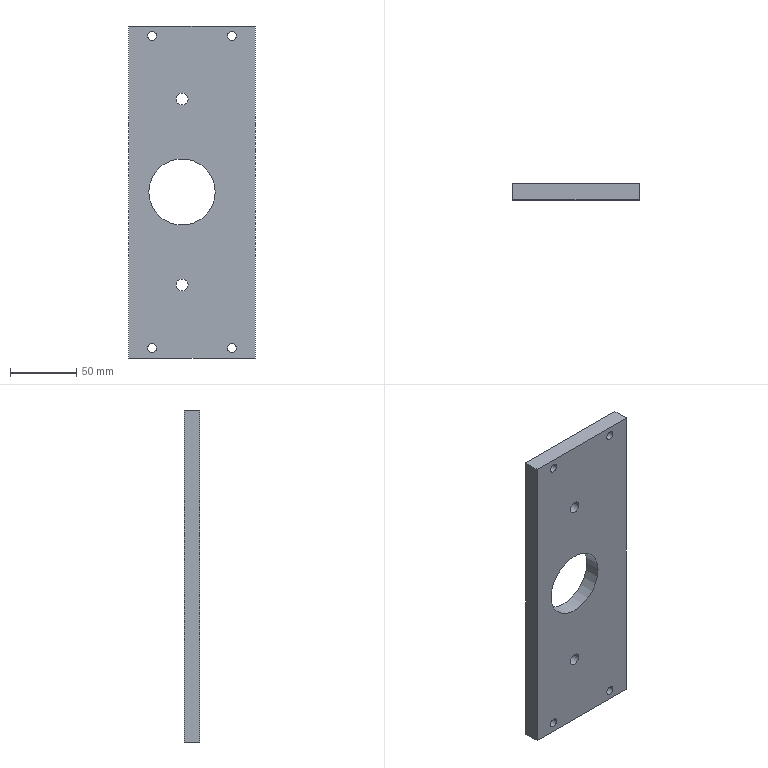Component | SolidWorks | 8TC-A15004-D0-03A-1 | 1 solid | 32 faces | box 95 x 12 x 250 mm | volume 256712 mm3 | cylinder 22 | plane 10 | commonest cylinder face diameters 11 x8 6.6 x8 9 x4 50 x2 | material #45
build123d program:
from build123d import *

# Parameters (mm, degrees)
SKETCH1_W                                       = 250
SKETCH1_H                                       = 95
BOSS_EXTRUDE1_DEPTH                             = 6
M8_CLEARANCE_HOLE_2_D                           = 9
M8_CLEARANCE_HOLE_1_D                           = 50
M6_HEX_SOCKET_HEAD_CAP_SCREW_CBORE1_D           = 6.6
M6_HEX_SOCKET_HEAD_CAP_SCREW_CBORE1_CBORE_D     = 11
M6_HEX_SOCKET_HEAD_CAP_SCREW_CBORE1_CBORE_DEPTH = 6.4


with BuildPart() as part:
    # Sketch1 → Boss-Extrude1 (new, symmetric)
    with BuildSketch(Plane(origin=(0, 0, 0), x_dir=(1, 0, 0), z_dir=(0, 1, 0))):
        Rectangle(SKETCH1_W, SKETCH1_H)
    extrude(amount=BOSS_EXTRUDE1_DEPTH, both=True)

    # M8 Clearance Hole 2 (through all)
    with Locations(Plane(origin=(0, -6, 0), x_dir=(-1, 0, 0), z_dir=(0, -1, 0))):
        with Locations((-70, -7.5), (70, -7.5)):
            Hole(M8_CLEARANCE_HOLE_2_D / 2)

    # M8 Clearance Hole 1 (through all)
    with Locations(Plane(origin=(0, -6, 0), x_dir=(-1, 0, 0), z_dir=(0, -1, 0))):
        with Locations((0, -7.5)):
            Hole(M8_CLEARANCE_HOLE_1_D / 2)

    # M6 Hex Socket Head Cap Screw CBORE1 (through all)
    with Locations(Plane(origin=(0, -6, 0), x_dir=(-1, 0, 0), z_dir=(0, -1, 0))):
        with Locations((-117.5, 30), (-117.5, -30), (117.5, 30), (117.5, -30)):
            CounterBoreHole(M6_HEX_SOCKET_HEAD_CAP_SCREW_CBORE1_D / 2, M6_HEX_SOCKET_HEAD_CAP_SCREW_CBORE1_CBORE_D / 2, M6_HEX_SOCKET_HEAD_CAP_SCREW_CBORE1_CBORE_DEPTH)


solid = part.part

# Placed as in the assembly
solid = solid.moved(Location((0, 428.5, 0), (180, -90, 0)))
STEP:
#1=CARTESIAN_POINT('',(0.9646,16.854,-4.626));
#2=VERTEX_POINT('',#1);
#3=CARTESIAN_POINT('',(1.398,16.854,-4.626));
#4=VERTEX_POINT('',#3);
#5=CARTESIAN_POINT('',(1.181,16.854,-4.626));
#6=DIRECTION('',(0.,1.,0.));
#7=DIRECTION('',(1.,0.,0.));
#8=AXIS2_PLACEMENT_3D('',#5,#6,#7);
#9=CIRCLE('',#8,0.2165);
#10=EDGE_CURVE('',#2,#4,#9,.T.);
#11=ORIENTED_EDGE('',*,*,#10,.F.);
#12=CARTESIAN_POINT('',(0.9646,17.106,-4.626));
#13=VERTEX_POINT('',#12);
#14=CARTESIAN_POINT('',(0.9646,17.106,-4.626));
#15=DIRECTION('',(0.,1.,0.));
#16=VECTOR('',#15,39.37);
#17=LINE('',#14,#16);
#18=EDGE_CURVE('',#2,#13,#17,.T.);
#19=ORIENTED_EDGE('',*,*,#18,.T.);
#20=CARTESIAN_POINT('',(1.398,17.106,-4.626));
#21=VERTEX_POINT('',#20);
#22=CARTESIAN_POINT('',(1.181,17.106,-4.626));
#23=DIRECTION('',(0.,1.,0.));
#24=DIRECTION('',(1.,0.,0.));
#25=AXIS2_PLACEMENT_3D('',#22,#23,#24);
#26=CIRCLE('',#25,0.2165);
#27=EDGE_CURVE('',#13,#21,#26,.T.);
#28=ORIENTED_EDGE('',*,*,#27,.T.);
#29=CARTESIAN_POINT('',(1.398,17.106,-4.626));
#30=DIRECTION('',(0.,1.,0.));
#31=VECTOR('',#30,39.37);
#32=LINE('',#29,#31);
#33=EDGE_CURVE('',#4,#21,#32,.T.);
#34=ORIENTED_EDGE('',*,*,#33,.F.);
#35=EDGE_LOOP('',(#11,#19,#28,#34));
#36=FACE_OUTER_BOUND('',#35,.T.);
#37=CARTESIAN_POINT('',(1.181,17.106,-4.626));
#38=DIRECTION('',(0.,1.,0.));
#39=DIRECTION('',(1.,0.,0.));
#40=AXIS2_PLACEMENT_3D('',#37,#38,#39);
#41=CYLINDRICAL_SURFACE('',#40,0.2165);
#42=ADVANCED_FACE('',(#36),#41,.F.);
#43=CARTESIAN_POINT('',(1.051,16.634,-4.626));
#44=VERTEX_POINT('',#43);
#45=CARTESIAN_POINT('',(1.311,16.634,-4.626));
#46=VERTEX_POINT('',#45);
#47=CARTESIAN_POINT('',(1.181,16.634,-4.626));
#48=DIRECTION('',(0.,1.,0.));
#49=DIRECTION('',(1.,0.,0.));
#50=AXIS2_PLACEMENT_3D('',#47,#48,#49);
#51=CIRCLE('',#50,0.1299);
#52=EDGE_CURVE('',#44,#46,#51,.T.);
#53=ORIENTED_EDGE('',*,*,#52,.F.);
#54=CARTESIAN_POINT('',(1.051,16.854,-4.626));
#55=VERTEX_POINT('',#54);
#56=CARTESIAN_POINT('',(1.051,17.106,-4.626));
#57=DIRECTION('',(0.,1.,0.));
#58=VECTOR('',#57,39.37);
#59=LINE('',#56,#58);
#60=EDGE_CURVE('',#44,#55,#59,.T.);
#61=ORIENTED_EDGE('',*,*,#60,.T.);
#62=CARTESIAN_POINT('',(1.311,16.854,-4.626));
#63=VERTEX_POINT('',#62);
#64=CARTESIAN_POINT('',(1.181,16.854,-4.626));
#65=DIRECTION('',(0.,1.,0.));
#66=DIRECTION('',(1.,0.,0.));
#67=AXIS2_PLACEMENT_3D('',#64,#65,#66);
#68=CIRCLE('',#67,0.1299);
#69=EDGE_CURVE('',#55,#63,#68,.T.);
#70=ORIENTED_EDGE('',*,*,#69,.T.);
#71=CARTESIAN_POINT('',(1.311,17.106,-4.626));
#72=DIRECTION('',(0.,1.,0.));
#73=VECTOR('',#72,39.37);
#74=LINE('',#71,#73);
#75=EDGE_CURVE('',#46,#63,#74,.T.);
#76=ORIENTED_EDGE('',*,*,#75,.F.);
#77=EDGE_LOOP('',(#53,#61,#70,#76));
#78=FACE_OUTER_BOUND('',#77,.T.);
#79=CARTESIAN_POINT('',(1.181,17.106,-4.626));
#80=DIRECTION('',(0.,1.,0.));
#81=DIRECTION('',(1.,0.,0.));
#82=AXIS2_PLACEMENT_3D('',#79,#80,#81);
#83=CYLINDRICAL_SURFACE('',#82,0.1299);
#84=ADVANCED_FACE('',(#78),#83,.F.);
#85=CARTESIAN_POINT('',(-1.398,16.854,-4.626));
#86=VERTEX_POINT('',#85);
#87=CARTESIAN_POINT('',(-0.9646,16.854,-4.626));
#88=VERTEX_POINT('',#87);
#89=CARTESIAN_POINT('',(-1.181,16.854,-4.626));
#90=DIRECTION('',(0.,1.,0.));
#91=DIRECTION('',(1.,0.,0.));
#92=AXIS2_PLACEMENT_3D('',#89,#90,#91);
#93=CIRCLE('',#92,0.2165);
#94=EDGE_CURVE('',#86,#88,#93,.T.);
#95=ORIENTED_EDGE('',*,*,#94,.F.);
#96=CARTESIAN_POINT('',(-1.398,17.106,-4.626));
#97=VERTEX_POINT('',#96);
#98=CARTESIAN_POINT('',(-1.398,17.106,-4.626));
#99=DIRECTION('',(0.,1.,0.));
#100=VECTOR('',#99,39.37);
#101=LINE('',#98,#100);
#102=EDGE_CURVE('',#86,#97,#101,.T.);
#103=ORIENTED_EDGE('',*,*,#102,.T.);
#104=CARTESIAN_POINT('',(-0.9646,17.106,-4.626));
#105=VERTEX_POINT('',#104);
#106=CARTESIAN_POINT('',(-1.181,17.106,-4.626));
#107=DIRECTION('',(0.,1.,0.));
#108=DIRECTION('',(1.,0.,0.));
#109=AXIS2_PLACEMENT_3D('',#106,#107,#108);
#110=CIRCLE('',#109,0.2165);
#111=EDGE_CURVE('',#97,#105,#110,.T.);
#112=ORIENTED_EDGE('',*,*,#111,.T.);
#113=CARTESIAN_POINT('',(-0.9646,17.106,-4.626));
#114=DIRECTION('',(0.,1.,0.));
#115=VECTOR('',#114,39.37);
#116=LINE('',#113,#115);
#117=EDGE_CURVE('',#88,#105,#116,.T.);
#118=ORIENTED_EDGE('',*,*,#117,.F.);
#119=EDGE_LOOP('',(#95,#103,#112,#118));
#120=FACE_OUTER_BOUND('',#119,.T.);
#121=CARTESIAN_POINT('',(-1.181,17.106,-4.626));
#122=DIRECTION('',(0.,1.,0.));
#123=DIRECTION('',(1.,0.,0.));
#124=AXIS2_PLACEMENT_3D('',#121,#122,#123);
#125=CYLINDRICAL_SURFACE('',#124,0.2165);
#126=ADVANCED_FACE('',(#120),#125,.F.);
#127=CARTESIAN_POINT('',(-1.311,16.634,-4.626));
#128=VERTEX_POINT('',#127);
#129=CARTESIAN_POINT('',(-1.051,16.634,-4.626));
#130=VERTEX_POINT('',#129);
#131=CARTESIAN_POINT('',(-1.181,16.634,-4.626));
#132=DIRECTION('',(0.,1.,0.));
#133=DIRECTION('',(1.,0.,0.));
#134=AXIS2_PLACEMENT_3D('',#131,#132,#133);
#135=CIRCLE('',#134,0.1299);
#136=EDGE_CURVE('',#128,#130,#135,.T.);
#137=ORIENTED_EDGE('',*,*,#136,.F.);
#138=CARTESIAN_POINT('',(-1.311,16.854,-4.626));
#139=VERTEX_POINT('',#138);
#140=CARTESIAN_POINT('',(-1.311,17.106,-4.626));
#141=DIRECTION('',(0.,1.,0.));
#142=VECTOR('',#141,39.37);
#143=LINE('',#140,#142);
#144=EDGE_CURVE('',#128,#139,#143,.T.);
#145=ORIENTED_EDGE('',*,*,#144,.T.);
#146=CARTESIAN_POINT('',(-1.051,16.854,-4.626));
#147=VERTEX_POINT('',#146);
#148=CARTESIAN_POINT('',(-1.181,16.854,-4.626));
#149=DIRECTION('',(0.,1.,0.));
#150=DIRECTION('',(1.,0.,0.));
#151=AXIS2_PLACEMENT_3D('',#148,#149,#150);
#152=CIRCLE('',#151,0.1299);
#153=EDGE_CURVE('',#139,#147,#152,.T.);
#154=ORIENTED_EDGE('',*,*,#153,.T.);
#155=CARTESIAN_POINT('',(-1.051,17.106,-4.626));
#156=DIRECTION('',(0.,1.,0.));
#157=VECTOR('',#156,39.37);
#158=LINE('',#155,#157);
#159=EDGE_CURVE('',#130,#147,#158,.T.);
#160=ORIENTED_EDGE('',*,*,#159,.F.);
#161=EDGE_LOOP('',(#137,#145,#154,#160));
#162=FACE_OUTER_BOUND('',#161,.T.);
#163=CARTESIAN_POINT('',(-1.181,17.106,-4.626));
#164=DIRECTION('',(0.,1.,0.));
#165=DIRECTION('',(1.,0.,0.));
#166=AXIS2_PLACEMENT_3D('',#163,#164,#165);
#167=CYLINDRICAL_SURFACE('',#166,0.1299);
#168=ADVANCED_FACE('',(#162),#167,.F.);
#169=CARTESIAN_POINT('',(0.9646,16.854,4.626));
#170=VERTEX_POINT('',#169);
#171=CARTESIAN_POINT('',(1.398,16.854,4.626));
#172=VERTEX_POINT('',#171);
#173=CARTESIAN_POINT('',(1.181,16.854,4.626));
#174=DIRECTION('',(0.,1.,0.));
#175=DIRECTION('',(1.,0.,0.));
#176=AXIS2_PLACEMENT_3D('',#173,#174,#175);
#177=CIRCLE('',#176,0.2165);
#178=EDGE_CURVE('',#170,#172,#177,.T.);
#179=ORIENTED_EDGE('',*,*,#178,.F.);
#180=CARTESIAN_POINT('',(0.9646,17.106,4.626));
#181=VERTEX_POINT('',#180);
#182=CARTESIAN_POINT('',(0.9646,17.106,4.626));
#183=DIRECTION('',(0.,1.,0.));
#184=VECTOR('',#183,39.37);
#185=LINE('',#182,#184);
#186=EDGE_CURVE('',#170,#181,#185,.T.);
#187=ORIENTED_EDGE('',*,*,#186,.T.);
#188=CARTESIAN_POINT('',(1.398,17.106,4.626));
#189=VERTEX_POINT('',#188);
#190=CARTESIAN_POINT('',(1.181,17.106,4.626));
#191=DIRECTION('',(0.,1.,0.));
#192=DIRECTION('',(1.,0.,0.));
#193=AXIS2_PLACEMENT_3D('',#190,#191,#192);
#194=CIRCLE('',#193,0.2165);
#195=EDGE_CURVE('',#181,#189,#194,.T.);
#196=ORIENTED_EDGE('',*,*,#195,.T.);
#197=CARTESIAN_POINT('',(1.398,17.106,4.626));
#198=DIRECTION('',(0.,1.,0.));
#199=VECTOR('',#198,39.37);
#200=LINE('',#197,#199);
#201=EDGE_CURVE('',#172,#189,#200,.T.);
#202=ORIENTED_EDGE('',*,*,#201,.F.);
#203=EDGE_LOOP('',(#179,#187,#196,#202));
#204=FACE_OUTER_BOUND('',#203,.T.);
#205=CARTESIAN_POINT('',(1.181,17.106,4.626));
#206=DIRECTION('',(0.,1.,0.));
#207=DIRECTION('',(1.,0.,0.));
#208=AXIS2_PLACEMENT_3D('',#205,#206,#207);
#209=CYLINDRICAL_SURFACE('',#208,0.2165);
#210=ADVANCED_FACE('',(#204),#209,.F.);
#211=CARTESIAN_POINT('',(1.051,16.634,4.626));
#212=VERTEX_POINT('',#211);
#213=CARTESIAN_POINT('',(1.311,16.634,4.626));
#214=VERTEX_POINT('',#213);
#215=CARTESIAN_POINT('',(1.181,16.634,4.626));
#216=DIRECTION('',(0.,1.,0.));
#217=DIRECTION('',(1.,0.,0.));
#218=AXIS2_PLACEMENT_3D('',#215,#216,#217);
#219=CIRCLE('',#218,0.1299);
#220=EDGE_CURVE('',#212,#214,#219,.T.);
#221=ORIENTED_EDGE('',*,*,#220,.F.);
#222=CARTESIAN_POINT('',(1.051,16.854,4.626));
#223=VERTEX_POINT('',#222);
#224=CARTESIAN_POINT('',(1.051,17.106,4.626));
#225=DIRECTION('',(0.,1.,0.));
#226=VECTOR('',#225,39.37);
#227=LINE('',#224,#226);
#228=EDGE_CURVE('',#212,#223,#227,.T.);
#229=ORIENTED_EDGE('',*,*,#228,.T.);
#230=CARTESIAN_POINT('',(1.311,16.854,4.626));
#231=VERTEX_POINT('',#230);
#232=CARTESIAN_POINT('',(1.181,16.854,4.626));
#233=DIRECTION('',(0.,1.,0.));
#234=DIRECTION('',(1.,0.,0.));
#235=AXIS2_PLACEMENT_3D('',#232,#233,#234);
#236=CIRCLE('',#235,0.1299);
#237=EDGE_CURVE('',#223,#231,#236,.T.);
#238=ORIENTED_EDGE('',*,*,#237,.T.);
#239=CARTESIAN_POINT('',(1.311,17.106,4.626));
#240=DIRECTION('',(0.,1.,0.));
#241=VECTOR('',#240,39.37);
#242=LINE('',#239,#241);
#243=EDGE_CURVE('',#214,#231,#242,.T.);
#244=ORIENTED_EDGE('',*,*,#243,.F.);
#245=EDGE_LOOP('',(#221,#229,#238,#244));
#246=FACE_OUTER_BOUND('',#245,.T.);
#247=CARTESIAN_POINT('',(1.181,17.106,4.626));
#248=DIRECTION('',(0.,1.,0.));
#249=DIRECTION('',(1.,0.,0.));
#250=AXIS2_PLACEMENT_3D('',#247,#248,#249);
#251=CYLINDRICAL_SURFACE('',#250,0.1299);
#252=ADVANCED_FACE('',(#246),#251,.F.);
#253=CARTESIAN_POINT('',(-1.398,16.854,4.626));
#254=VERTEX_POINT('',#253);
#255=CARTESIAN_POINT('',(-0.9646,16.854,4.626));
#256=VERTEX_POINT('',#255);
#257=CARTESIAN_POINT('',(-1.181,16.854,4.626));
#258=DIRECTION('',(0.,1.,0.));
#259=DIRECTION('',(1.,0.,0.));
#260=AXIS2_PLACEMENT_3D('',#257,#258,#259);
#261=CIRCLE('',#260,0.2165);
#262=EDGE_CURVE('',#254,#256,#261,.T.);
#263=ORIENTED_EDGE('',*,*,#262,.F.);
#264=CARTESIAN_POINT('',(-1.398,17.106,4.626));
#265=VERTEX_POINT('',#264);
#266=CARTESIAN_POINT('',(-1.398,17.106,4.626));
#267=DIRECTION('',(0.,1.,0.));
#268=VECTOR('',#267,39.37);
#269=LINE('',#266,#268);
#270=EDGE_CURVE('',#254,#265,#269,.T.);
#271=ORIENTED_EDGE('',*,*,#270,.T.);
#272=CARTESIAN_POINT('',(-0.9646,17.106,4.626));
#273=VERTEX_POINT('',#272);
#274=CARTESIAN_POINT('',(-1.181,17.106,4.626));
#275=DIRECTION('',(0.,1.,0.));
#276=DIRECTION('',(1.,0.,0.));
#277=AXIS2_PLACEMENT_3D('',#274,#275,#276);
#278=CIRCLE('',#277,0.2165);
#279=EDGE_CURVE('',#265,#273,#278,.T.);
#280=ORIENTED_EDGE('',*,*,#279,.T.);
#281=CARTESIAN_POINT('',(-0.9646,17.106,4.626));
#282=DIRECTION('',(0.,1.,0.));
#283=VECTOR('',#282,39.37);
#284=LINE('',#281,#283);
#285=EDGE_CURVE('',#256,#273,#284,.T.);
#286=ORIENTED_EDGE('',*,*,#285,.F.);
#287=EDGE_LOOP('',(#263,#271,#280,#286));
#288=FACE_OUTER_BOUND('',#287,.T.);
#289=CARTESIAN_POINT('',(-1.181,17.106,4.626));
#290=DIRECTION('',(0.,1.,0.));
#291=DIRECTION('',(1.,0.,0.));
#292=AXIS2_PLACEMENT_3D('',#289,#290,#291);
#293=CYLINDRICAL_SURFACE('',#292,0.2165);
#294=ADVANCED_FACE('',(#288),#293,.F.);
#295=CARTESIAN_POINT('',(-1.311,16.634,4.626));
#296=VERTEX_POINT('',#295);
#297=CARTESIAN_POINT('',(-1.051,16.634,4.626));
#298=VERTEX_POINT('',#297);
#299=CARTESIAN_POINT('',(-1.181,16.634,4.626));
#300=DIRECTION('',(0.,1.,0.));
#301=DIRECTION('',(1.,0.,0.));
#302=AXIS2_PLACEMENT_3D('',#299,#300,#301);
#303=CIRCLE('',#302,0.1299);
#304=EDGE_CURVE('',#296,#298,#303,.T.);
#305=ORIENTED_EDGE('',*,*,#304,.F.);
#306=CARTESIAN_POINT('',(-1.311,16.854,4.626));
#307=VERTEX_POINT('',#306);
#308=CARTESIAN_POINT('',(-1.311,17.106,4.626));
#309=DIRECTION('',(0.,1.,0.));
#310=VECTOR('',#309,39.37);
#311=LINE('',#308,#310);
#312=EDGE_CURVE('',#296,#307,#311,.T.);
#313=ORIENTED_EDGE('',*,*,#312,.T.);
#314=CARTESIAN_POINT('',(-1.051,16.854,4.626));
#315=VERTEX_POINT('',#314);
#316=CARTESIAN_POINT('',(-1.181,16.854,4.626));
#317=DIRECTION('',(0.,1.,0.));
#318=DIRECTION('',(1.,0.,0.));
#319=AXIS2_PLACEMENT_3D('',#316,#317,#318);
#320=CIRCLE('',#319,0.1299);
#321=EDGE_CURVE('',#307,#315,#320,.T.);
#322=ORIENTED_EDGE('',*,*,#321,.T.);
#323=CARTESIAN_POINT('',(-1.051,17.106,4.626));
#324=DIRECTION('',(0.,1.,0.));
#325=VECTOR('',#324,39.37);
#326=LINE('',#323,#325);
#327=EDGE_CURVE('',#298,#315,#326,.T.);
#328=ORIENTED_EDGE('',*,*,#327,.F.);
#329=EDGE_LOOP('',(#305,#313,#322,#328));
#330=FACE_OUTER_BOUND('',#329,.T.);
#331=CARTESIAN_POINT('',(-1.181,17.106,4.626));
#332=DIRECTION('',(0.,1.,0.));
#333=DIRECTION('',(1.,0.,0.));
#334=AXIS2_PLACEMENT_3D('',#331,#332,#333);
#335=CYLINDRICAL_SURFACE('',#334,0.1299);
#336=ADVANCED_FACE('',(#330),#335,.F.);
#337=CARTESIAN_POINT('',(-1.28,16.634,-0.));
#338=VERTEX_POINT('',#337);
#339=CARTESIAN_POINT('',(0.689,16.634,-0.));
#340=VERTEX_POINT('',#339);
#341=CARTESIAN_POINT('',(-0.2953,16.634,-0.));
#342=DIRECTION('',(0.,1.,0.));
#343=DIRECTION('',(1.,0.,-0.));
#344=AXIS2_PLACEMENT_3D('',#341,#342,#343);
#345=CIRCLE('',#344,0.9843);
#346=EDGE_CURVE('',#338,#340,#345,.T.);
#347=ORIENTED_EDGE('',*,*,#346,.F.);
#348=CARTESIAN_POINT('',(-1.28,17.106,-0.));
#349=VERTEX_POINT('',#348);
#350=CARTESIAN_POINT('',(-1.28,17.106,-0.));
#351=DIRECTION('',(0.,1.,0.));
#352=VECTOR('',#351,39.37);
#353=LINE('',#350,#352);
#354=EDGE_CURVE('',#338,#349,#353,.T.);
#355=ORIENTED_EDGE('',*,*,#354,.T.);
#356=CARTESIAN_POINT('',(0.689,17.106,-0.));
#357=VERTEX_POINT('',#356);
#358=CARTESIAN_POINT('',(-0.2953,17.106,-0.));
#359=DIRECTION('',(0.,1.,0.));
#360=DIRECTION('',(1.,0.,-0.));
#361=AXIS2_PLACEMENT_3D('',#358,#359,#360);
#362=CIRCLE('',#361,0.9843);
#363=EDGE_CURVE('',#349,#357,#362,.T.);
#364=ORIENTED_EDGE('',*,*,#363,.T.);
#365=CARTESIAN_POINT('',(0.689,17.106,-0.));
#366=DIRECTION('',(0.,1.,0.));
#367=VECTOR('',#366,39.37);
#368=LINE('',#365,#367);
#369=EDGE_CURVE('',#340,#357,#368,.T.);
#370=ORIENTED_EDGE('',*,*,#369,.F.);
#371=EDGE_LOOP('',(#347,#355,#364,#370));
#372=FACE_OUTER_BOUND('',#371,.T.);
#373=CARTESIAN_POINT('',(-0.2953,17.106,-0.));
#374=DIRECTION('',(0.,1.,0.));
#375=DIRECTION('',(1.,0.,-0.));
#376=AXIS2_PLACEMENT_3D('',#373,#374,#375);
#377=CYLINDRICAL_SURFACE('',#376,0.9843);
#378=ADVANCED_FACE('',(#372),#377,.F.);
#379=CARTESIAN_POINT('',(-0.4724,16.634,-2.756));
#380=VERTEX_POINT('',#379);
#381=CARTESIAN_POINT('',(-0.1181,16.634,-2.756));
#382=VERTEX_POINT('',#381);
#383=CARTESIAN_POINT('',(-0.2953,16.634,-2.756));
#384=DIRECTION('',(0.,1.,0.));
#385=DIRECTION('',(1.,0.,0.));
#386=AXIS2_PLACEMENT_3D('',#383,#384,#385);
#387=CIRCLE('',#386,0.1772);
#388=EDGE_CURVE('',#380,#382,#387,.T.);
#389=ORIENTED_EDGE('',*,*,#388,.F.);
#390=CARTESIAN_POINT('',(-0.4724,17.106,-2.756));
#391=VERTEX_POINT('',#390);
#392=CARTESIAN_POINT('',(-0.4724,17.106,-2.756));
#393=DIRECTION('',(0.,1.,0.));
#394=VECTOR('',#393,39.37);
#395=LINE('',#392,#394);
#396=EDGE_CURVE('',#380,#391,#395,.T.);
#397=ORIENTED_EDGE('',*,*,#396,.T.);
#398=CARTESIAN_POINT('',(-0.1181,17.106,-2.756));
#399=VERTEX_POINT('',#398);
#400=CARTESIAN_POINT('',(-0.2953,17.106,-2.756));
#401=DIRECTION('',(0.,1.,0.));
#402=DIRECTION('',(1.,0.,0.));
#403=AXIS2_PLACEMENT_3D('',#400,#401,#402);
#404=CIRCLE('',#403,0.1772);
#405=EDGE_CURVE('',#391,#399,#404,.T.);
#406=ORIENTED_EDGE('',*,*,#405,.T.);
#407=CARTESIAN_POINT('',(-0.1181,17.106,-2.756));
#408=DIRECTION('',(0.,1.,0.));
#409=VECTOR('',#408,39.37);
#410=LINE('',#407,#409);
#411=EDGE_CURVE('',#382,#399,#410,.T.);
#412=ORIENTED_EDGE('',*,*,#411,.F.);
#413=EDGE_LOOP('',(#389,#397,#406,#412));
#414=FACE_OUTER_BOUND('',#413,.T.);
#415=CARTESIAN_POINT('',(-0.2953,17.106,-2.756));
#416=DIRECTION('',(0.,1.,0.));
#417=DIRECTION('',(1.,0.,0.));
#418=AXIS2_PLACEMENT_3D('',#415,#416,#417);
#419=CYLINDRICAL_SURFACE('',#418,0.1772);
#420=ADVANCED_FACE('',(#414),#419,.F.);
#421=CARTESIAN_POINT('',(-0.4724,16.634,2.756));
#422=VERTEX_POINT('',#421);
#423=CARTESIAN_POINT('',(-0.1181,16.634,2.756));
#424=VERTEX_POINT('',#423);
#425=CARTESIAN_POINT('',(-0.2953,16.634,2.756));
#426=DIRECTION('',(0.,1.,0.));
#427=DIRECTION('',(1.,0.,0.));
#428=AXIS2_PLACEMENT_3D('',#425,#426,#427);
#429=CIRCLE('',#428,0.1772);
#430=EDGE_CURVE('',#422,#424,#429,.T.);
#431=ORIENTED_EDGE('',*,*,#430,.F.);
#432=CARTESIAN_POINT('',(-0.4724,17.106,2.756));
#433=VERTEX_POINT('',#432);
#434=CARTESIAN_POINT('',(-0.4724,17.106,2.756));
#435=DIRECTION('',(0.,1.,0.));
#436=VECTOR('',#435,39.37);
#437=LINE('',#434,#436);
#438=EDGE_CURVE('',#422,#433,#437,.T.);
#439=ORIENTED_EDGE('',*,*,#438,.T.);
#440=CARTESIAN_POINT('',(-0.1181,17.106,2.756));
#441=VERTEX_POINT('',#440);
#442=CARTESIAN_POINT('',(-0.2953,17.106,2.756));
#443=DIRECTION('',(0.,1.,0.));
#444=DIRECTION('',(1.,0.,0.));
#445=AXIS2_PLACEMENT_3D('',#442,#443,#444);
#446=CIRCLE('',#445,0.1772);
#447=EDGE_CURVE('',#433,#441,#446,.T.);
#448=ORIENTED_EDGE('',*,*,#447,.T.);
#449=CARTESIAN_POINT('',(-0.1181,17.106,2.756));
#450=DIRECTION('',(0.,1.,0.));
#451=VECTOR('',#450,39.37);
#452=LINE('',#449,#451);
#453=EDGE_CURVE('',#424,#441,#452,.T.);
#454=ORIENTED_EDGE('',*,*,#453,.F.);
#455=EDGE_LOOP('',(#431,#439,#448,#454));
#456=FACE_OUTER_BOUND('',#455,.T.);
#457=CARTESIAN_POINT('',(-0.2953,17.106,2.756));
#458=DIRECTION('',(0.,1.,0.));
#459=DIRECTION('',(1.,0.,0.));
#460=AXIS2_PLACEMENT_3D('',#457,#458,#459);
#461=CYLINDRICAL_SURFACE('',#460,0.1772);
#462=ADVANCED_FACE('',(#456),#461,.F.);
#463=CARTESIAN_POINT('',(-1.87,17.106,-4.921));
#464=VERTEX_POINT('',#463);
#465=CARTESIAN_POINT('',(1.87,17.106,-4.921));
#466=VERTEX_POINT('',#465);
#467=CARTESIAN_POINT('',(-1.87,17.106,-4.921));
#468=DIRECTION('',(1.,0.,-0.));
#469=VECTOR('',#468,39.37);
#470=LINE('',#467,#469);
#471=EDGE_CURVE('',#464,#466,#470,.T.);
#472=ORIENTED_EDGE('',*,*,#471,.T.);
#473=CARTESIAN_POINT('',(1.87,16.634,-4.921));
#474=VERTEX_POINT('',#473);
#475=CARTESIAN_POINT('',(1.87,16.634,-4.921));
#476=DIRECTION('',(0.,1.,0.));
#477=VECTOR('',#476,39.37);
#478=LINE('',#475,#477);
#479=EDGE_CURVE('',#474,#466,#478,.T.);
#480=ORIENTED_EDGE('',*,*,#479,.F.);
#481=CARTESIAN_POINT('',(-1.87,16.634,-4.921));
#482=VERTEX_POINT('',#481);
#483=CARTESIAN_POINT('',(-1.87,16.634,-4.921));
#484=DIRECTION('',(1.,0.,-0.));
#485=VECTOR('',#484,39.37);
#486=LINE('',#483,#485);
#487=EDGE_CURVE('',#482,#474,#486,.T.);
#488=ORIENTED_EDGE('',*,*,#487,.F.);
#489=CARTESIAN_POINT('',(-1.87,16.634,-4.921));
#490=DIRECTION('',(0.,1.,0.));
#491=VECTOR('',#490,39.37);
#492=LINE('',#489,#491);
#493=EDGE_CURVE('',#482,#464,#492,.T.);
#494=ORIENTED_EDGE('',*,*,#493,.T.);
#495=EDGE_LOOP('',(#472,#480,#488,#494));
#496=FACE_OUTER_BOUND('',#495,.T.);
#497=CARTESIAN_POINT('',(-1.87,16.634,-4.921));
#498=DIRECTION('',(0.,0.,1.));
#499=DIRECTION('',(-1.,0.,0.));
#500=AXIS2_PLACEMENT_3D('',#497,#498,#499);
#501=PLANE('',#500);
#502=ADVANCED_FACE('',(#496),#501,.F.);
#503=CARTESIAN_POINT('',(1.87,17.106,4.921));
#504=VERTEX_POINT('',#503);
#505=CARTESIAN_POINT('',(1.87,17.106,4.921));
#506=DIRECTION('',(0.,0.,1.));
#507=VECTOR('',#506,39.37);
#508=LINE('',#505,#507);
#509=EDGE_CURVE('',#466,#504,#508,.T.);
#510=ORIENTED_EDGE('',*,*,#509,.T.);
#511=CARTESIAN_POINT('',(1.87,16.634,4.921));
#512=VERTEX_POINT('',#511);
#513=CARTESIAN_POINT('',(1.87,16.634,4.921));
#514=DIRECTION('',(0.,1.,0.));
#515=VECTOR('',#514,39.37);
#516=LINE('',#513,#515);
#517=EDGE_CURVE('',#512,#504,#516,.T.);
#518=ORIENTED_EDGE('',*,*,#517,.F.);
#519=CARTESIAN_POINT('',(1.87,16.634,4.921));
#520=DIRECTION('',(0.,0.,1.));
#521=VECTOR('',#520,39.37);
#522=LINE('',#519,#521);
#523=EDGE_CURVE('',#474,#512,#522,.T.);
#524=ORIENTED_EDGE('',*,*,#523,.F.);
#525=ORIENTED_EDGE('',*,*,#479,.T.);
#526=EDGE_LOOP('',(#510,#518,#524,#525));
#527=FACE_OUTER_BOUND('',#526,.T.);
#528=CARTESIAN_POINT('',(1.87,16.634,4.921));
#529=DIRECTION('',(-1.,0.,0.));
#530=DIRECTION('',(-0.,0.,-1.));
#531=AXIS2_PLACEMENT_3D('',#528,#529,#530);
#532=PLANE('',#531);
#533=ADVANCED_FACE('',(#527),#532,.F.);
#534=CARTESIAN_POINT('',(-1.87,17.106,4.921));
#535=VERTEX_POINT('',#534);
#536=CARTESIAN_POINT('',(-1.87,17.106,4.921));
#537=DIRECTION('',(-1.,0.,0.));
#538=VECTOR('',#537,39.37);
#539=LINE('',#536,#538);
#540=EDGE_CURVE('',#504,#535,#539,.T.);
#541=ORIENTED_EDGE('',*,*,#540,.T.);
#542=CARTESIAN_POINT('',(-1.87,16.634,4.921));
#543=VERTEX_POINT('',#542);
#544=CARTESIAN_POINT('',(-1.87,16.634,4.921));
#545=DIRECTION('',(0.,1.,0.));
#546=VECTOR('',#545,39.37);
#547=LINE('',#544,#546);
#548=EDGE_CURVE('',#543,#535,#547,.T.);
#549=ORIENTED_EDGE('',*,*,#548,.F.);
#550=CARTESIAN_POINT('',(-1.87,16.634,4.921));
#551=DIRECTION('',(-1.,0.,0.));
#552=VECTOR('',#551,39.37);
#553=LINE('',#550,#552);
#554=EDGE_CURVE('',#512,#543,#553,.T.);
#555=ORIENTED_EDGE('',*,*,#554,.F.);
#556=ORIENTED_EDGE('',*,*,#517,.T.);
#557=EDGE_LOOP('',(#541,#549,#555,#556));
#558=FACE_OUTER_BOUND('',#557,.T.);
#559=CARTESIAN_POINT('',(-1.87,16.634,4.921));
#560=DIRECTION('',(-0.,0.,-1.));
#561=DIRECTION('',(1.,0.,-0.));
#562=AXIS2_PLACEMENT_3D('',#559,#560,#561);
#563=PLANE('',#562);
#564=ADVANCED_FACE('',(#558),#563,.F.);
#565=CARTESIAN_POINT('',(-1.87,17.106,4.921));
#566=DIRECTION('',(-0.,0.,-1.));
#567=VECTOR('',#566,39.37);
#568=LINE('',#565,#567);
#569=EDGE_CURVE('',#535,#464,#568,.T.);
#570=ORIENTED_EDGE('',*,*,#569,.T.);
#571=ORIENTED_EDGE('',*,*,#493,.F.);
#572=CARTESIAN_POINT('',(-1.87,16.634,4.921));
#573=DIRECTION('',(-0.,0.,-1.));
#574=VECTOR('',#573,39.37);
#575=LINE('',#572,#574);
#576=EDGE_CURVE('',#543,#482,#575,.T.);
#577=ORIENTED_EDGE('',*,*,#576,.F.);
#578=ORIENTED_EDGE('',*,*,#548,.T.);
#579=EDGE_LOOP('',(#570,#571,#577,#578));
#580=FACE_OUTER_BOUND('',#579,.T.);
#581=CARTESIAN_POINT('',(-1.87,16.634,4.921));
#582=DIRECTION('',(1.,0.,-0.));
#583=DIRECTION('',(0.,0.,1.));
#584=AXIS2_PLACEMENT_3D('',#581,#582,#583);
#585=PLANE('',#584);
#586=ADVANCED_FACE('',(#580),#585,.F.);
#587=CARTESIAN_POINT('',(1.181,16.634,-4.626));
#588=DIRECTION('',(0.,1.,0.));
#589=DIRECTION('',(1.,0.,0.));
#590=AXIS2_PLACEMENT_3D('',#587,#588,#589);
#591=CIRCLE('',#590,0.1299);
#592=EDGE_CURVE('',#46,#44,#591,.T.);
#593=ORIENTED_EDGE('',*,*,#592,.T.);
#594=ORIENTED_EDGE('',*,*,#52,.T.);
#595=EDGE_LOOP('',(#593,#594));
#596=FACE_BOUND('',#595,.T.);
#597=CARTESIAN_POINT('',(-1.181,16.634,-4.626));
#598=DIRECTION('',(0.,1.,0.));
#599=DIRECTION('',(1.,0.,0.));
#600=AXIS2_PLACEMENT_3D('',#597,#598,#599);
#601=CIRCLE('',#600,0.1299);
#602=EDGE_CURVE('',#130,#128,#601,.T.);
#603=ORIENTED_EDGE('',*,*,#602,.T.);
#604=ORIENTED_EDGE('',*,*,#136,.T.);
#605=EDGE_LOOP('',(#603,#604));
#606=FACE_BOUND('',#605,.T.);
#607=CARTESIAN_POINT('',(1.181,16.634,4.626));
#608=DIRECTION('',(0.,1.,0.));
#609=DIRECTION('',(1.,0.,0.));
#610=AXIS2_PLACEMENT_3D('',#607,#608,#609);
#611=CIRCLE('',#610,0.1299);
#612=EDGE_CURVE('',#214,#212,#611,.T.);
#613=ORIENTED_EDGE('',*,*,#612,.T.);
#614=ORIENTED_EDGE('',*,*,#220,.T.);
#615=EDGE_LOOP('',(#613,#614));
#616=FACE_BOUND('',#615,.T.);
#617=CARTESIAN_POINT('',(-1.181,16.634,4.626));
#618=DIRECTION('',(0.,1.,0.));
#619=DIRECTION('',(1.,0.,0.));
#620=AXIS2_PLACEMENT_3D('',#617,#618,#619);
#621=CIRCLE('',#620,0.1299);
#622=EDGE_CURVE('',#298,#296,#621,.T.);
#623=ORIENTED_EDGE('',*,*,#622,.T.);
#624=ORIENTED_EDGE('',*,*,#304,.T.);
#625=EDGE_LOOP('',(#623,#624));
#626=FACE_BOUND('',#625,.T.);
#627=CARTESIAN_POINT('',(-0.2953,16.634,-0.));
#628=DIRECTION('',(0.,1.,0.));
#629=DIRECTION('',(1.,0.,-0.));
#630=AXIS2_PLACEMENT_3D('',#627,#628,#629);
#631=CIRCLE('',#630,0.9843);
#632=EDGE_CURVE('',#340,#338,#631,.T.);
#633=ORIENTED_EDGE('',*,*,#632,.T.);
#634=ORIENTED_EDGE('',*,*,#346,.T.);
#635=EDGE_LOOP('',(#633,#634));
#636=FACE_BOUND('',#635,.T.);
#637=CARTESIAN_POINT('',(-0.2953,16.634,-2.756));
#638=DIRECTION('',(0.,1.,0.));
#639=DIRECTION('',(1.,0.,0.));
#640=AXIS2_PLACEMENT_3D('',#637,#638,#639);
#641=CIRCLE('',#640,0.1772);
#642=EDGE_CURVE('',#382,#380,#641,.T.);
#643=ORIENTED_EDGE('',*,*,#642,.T.);
#644=ORIENTED_EDGE('',*,*,#388,.T.);
#645=EDGE_LOOP('',(#643,#644));
#646=FACE_BOUND('',#645,.T.);
#647=CARTESIAN_POINT('',(-0.2953,16.634,2.756));
#648=DIRECTION('',(0.,1.,0.));
#649=DIRECTION('',(1.,0.,0.));
#650=AXIS2_PLACEMENT_3D('',#647,#648,#649);
#651=CIRCLE('',#650,0.1772);
#652=EDGE_CURVE('',#424,#422,#651,.T.);
#653=ORIENTED_EDGE('',*,*,#652,.T.);
#654=ORIENTED_EDGE('',*,*,#430,.T.);
#655=EDGE_LOOP('',(#653,#654));
#656=FACE_BOUND('',#655,.T.);
#657=ORIENTED_EDGE('',*,*,#487,.T.);
#658=ORIENTED_EDGE('',*,*,#523,.T.);
#659=ORIENTED_EDGE('',*,*,#554,.T.);
#660=ORIENTED_EDGE('',*,*,#576,.T.);
#661=EDGE_LOOP('',(#657,#658,#659,#660));
#662=FACE_OUTER_BOUND('',#661,.T.);
#663=CARTESIAN_POINT('',(-0.,16.634,-0.));
#664=DIRECTION('',(0.,1.,0.));
#665=DIRECTION('',(1.,0.,-0.));
#666=AXIS2_PLACEMENT_3D('',#663,#664,#665);
#667=PLANE('',#666);
#668=ADVANCED_FACE('',(#596,#606,#616,#626,#636,#646,#656,#662),#667,.F.);
#669=CARTESIAN_POINT('',(1.181,17.106,-4.626));
#670=DIRECTION('',(0.,1.,0.));
#671=DIRECTION('',(1.,0.,0.));
#672=AXIS2_PLACEMENT_3D('',#669,#670,#671);
#673=CIRCLE('',#672,0.2165);
#674=EDGE_CURVE('',#21,#13,#673,.T.);
#675=ORIENTED_EDGE('',*,*,#674,.F.);
#676=ORIENTED_EDGE('',*,*,#27,.F.);
#677=EDGE_LOOP('',(#675,#676));
#678=FACE_BOUND('',#677,.T.);
#679=CARTESIAN_POINT('',(-1.181,17.106,-4.626));
#680=DIRECTION('',(0.,1.,0.));
#681=DIRECTION('',(1.,0.,0.));
#682=AXIS2_PLACEMENT_3D('',#679,#680,#681);
#683=CIRCLE('',#682,0.2165);
#684=EDGE_CURVE('',#105,#97,#683,.T.);
#685=ORIENTED_EDGE('',*,*,#684,.F.);
#686=ORIENTED_EDGE('',*,*,#111,.F.);
#687=EDGE_LOOP('',(#685,#686));
#688=FACE_BOUND('',#687,.T.);
#689=CARTESIAN_POINT('',(1.181,17.106,4.626));
#690=DIRECTION('',(0.,1.,0.));
#691=DIRECTION('',(1.,0.,0.));
#692=AXIS2_PLACEMENT_3D('',#689,#690,#691);
#693=CIRCLE('',#692,0.2165);
#694=EDGE_CURVE('',#189,#181,#693,.T.);
#695=ORIENTED_EDGE('',*,*,#694,.F.);
#696=ORIENTED_EDGE('',*,*,#195,.F.);
#697=EDGE_LOOP('',(#695,#696));
#698=FACE_BOUND('',#697,.T.);
#699=CARTESIAN_POINT('',(-1.181,17.106,4.626));
#700=DIRECTION('',(0.,1.,0.));
#701=DIRECTION('',(1.,0.,0.));
#702=AXIS2_PLACEMENT_3D('',#699,#700,#701);
#703=CIRCLE('',#702,0.2165);
#704=EDGE_CURVE('',#273,#265,#703,.T.);
#705=ORIENTED_EDGE('',*,*,#704,.F.);
#706=ORIENTED_EDGE('',*,*,#279,.F.);
#707=EDGE_LOOP('',(#705,#706));
#708=FACE_BOUND('',#707,.T.);
#709=CARTESIAN_POINT('',(-0.2953,17.106,-0.));
#710=DIRECTION('',(0.,1.,0.));
#711=DIRECTION('',(1.,0.,-0.));
#712=AXIS2_PLACEMENT_3D('',#709,#710,#711);
#713=CIRCLE('',#712,0.9843);
#714=EDGE_CURVE('',#357,#349,#713,.T.);
#715=ORIENTED_EDGE('',*,*,#714,.F.);
#716=ORIENTED_EDGE('',*,*,#363,.F.);
#717=EDGE_LOOP('',(#715,#716));
#718=FACE_BOUND('',#717,.T.);
#719=CARTESIAN_POINT('',(-0.2953,17.106,-2.756));
#720=DIRECTION('',(0.,1.,0.));
#721=DIRECTION('',(1.,0.,0.));
#722=AXIS2_PLACEMENT_3D('',#719,#720,#721);
#723=CIRCLE('',#722,0.1772);
#724=EDGE_CURVE('',#399,#391,#723,.T.);
#725=ORIENTED_EDGE('',*,*,#724,.F.);
#726=ORIENTED_EDGE('',*,*,#405,.F.);
#727=EDGE_LOOP('',(#725,#726));
#728=FACE_BOUND('',#727,.T.);
#729=CARTESIAN_POINT('',(-0.2953,17.106,2.756));
#730=DIRECTION('',(0.,1.,0.));
#731=DIRECTION('',(1.,0.,0.));
#732=AXIS2_PLACEMENT_3D('',#729,#730,#731);
#733=CIRCLE('',#732,0.1772);
#734=EDGE_CURVE('',#441,#433,#733,.T.);
#735=ORIENTED_EDGE('',*,*,#734,.F.);
#736=ORIENTED_EDGE('',*,*,#447,.F.);
#737=EDGE_LOOP('',(#735,#736));
#738=FACE_BOUND('',#737,.T.);
#739=ORIENTED_EDGE('',*,*,#471,.F.);
#740=ORIENTED_EDGE('',*,*,#569,.F.);
#741=ORIENTED_EDGE('',*,*,#540,.F.);
#742=ORIENTED_EDGE('',*,*,#509,.F.);
#743=EDGE_LOOP('',(#739,#740,#741,#742));
#744=FACE_OUTER_BOUND('',#743,.T.);
#745=CARTESIAN_POINT('',(-0.,17.106,-0.));
#746=DIRECTION('',(0.,1.,0.));
#747=DIRECTION('',(1.,0.,-0.));
#748=AXIS2_PLACEMENT_3D('',#745,#746,#747);
#749=PLANE('',#748);
#750=ADVANCED_FACE('',(#678,#688,#698,#708,#718,#728,#738,#744),#749,.T.);
#751=ORIENTED_EDGE('',*,*,#438,.F.);
#752=ORIENTED_EDGE('',*,*,#652,.F.);
#753=ORIENTED_EDGE('',*,*,#453,.T.);
#754=ORIENTED_EDGE('',*,*,#734,.T.);
#755=EDGE_LOOP('',(#751,#752,#753,#754));
#756=FACE_OUTER_BOUND('',#755,.T.);
#757=CARTESIAN_POINT('',(-0.2953,17.106,2.756));
#758=DIRECTION('',(0.,1.,0.));
#759=DIRECTION('',(1.,0.,0.));
#760=AXIS2_PLACEMENT_3D('',#757,#758,#759);
#761=CYLINDRICAL_SURFACE('',#760,0.1772);
#762=ADVANCED_FACE('',(#756),#761,.F.);
#763=ORIENTED_EDGE('',*,*,#396,.F.);
#764=ORIENTED_EDGE('',*,*,#642,.F.);
#765=ORIENTED_EDGE('',*,*,#411,.T.);
#766=ORIENTED_EDGE('',*,*,#724,.T.);
#767=EDGE_LOOP('',(#763,#764,#765,#766));
#768=FACE_OUTER_BOUND('',#767,.T.);
#769=CARTESIAN_POINT('',(-0.2953,17.106,-2.756));
#770=DIRECTION('',(0.,1.,0.));
#771=DIRECTION('',(1.,0.,0.));
#772=AXIS2_PLACEMENT_3D('',#769,#770,#771);
#773=CYLINDRICAL_SURFACE('',#772,0.1772);
#774=ADVANCED_FACE('',(#768),#773,.F.);
#775=ORIENTED_EDGE('',*,*,#354,.F.);
#776=ORIENTED_EDGE('',*,*,#632,.F.);
#777=ORIENTED_EDGE('',*,*,#369,.T.);
#778=ORIENTED_EDGE('',*,*,#714,.T.);
#779=EDGE_LOOP('',(#775,#776,#777,#778));
#780=FACE_OUTER_BOUND('',#779,.T.);
#781=CARTESIAN_POINT('',(-0.2953,17.106,-0.));
#782=DIRECTION('',(0.,1.,0.));
#783=DIRECTION('',(1.,0.,-0.));
#784=AXIS2_PLACEMENT_3D('',#781,#782,#783);
#785=CYLINDRICAL_SURFACE('',#784,0.9843);
#786=ADVANCED_FACE('',(#780),#785,.F.);
#787=ORIENTED_EDGE('',*,*,#312,.F.);
#788=ORIENTED_EDGE('',*,*,#622,.F.);
#789=ORIENTED_EDGE('',*,*,#327,.T.);
#790=CARTESIAN_POINT('',(-1.181,16.854,4.626));
#791=DIRECTION('',(0.,1.,0.));
#792=DIRECTION('',(1.,0.,0.));
#793=AXIS2_PLACEMENT_3D('',#790,#791,#792);
#794=CIRCLE('',#793,0.1299);
#795=EDGE_CURVE('',#315,#307,#794,.T.);
#796=ORIENTED_EDGE('',*,*,#795,.T.);
#797=EDGE_LOOP('',(#787,#788,#789,#796));
#798=FACE_OUTER_BOUND('',#797,.T.);
#799=CARTESIAN_POINT('',(-1.181,17.106,4.626));
#800=DIRECTION('',(0.,1.,0.));
#801=DIRECTION('',(1.,0.,0.));
#802=AXIS2_PLACEMENT_3D('',#799,#800,#801);
#803=CYLINDRICAL_SURFACE('',#802,0.1299);
#804=ADVANCED_FACE('',(#798),#803,.F.);
#805=ORIENTED_EDGE('',*,*,#795,.F.);
#806=ORIENTED_EDGE('',*,*,#321,.F.);
#807=EDGE_LOOP('',(#805,#806));
#808=FACE_BOUND('',#807,.T.);
#809=CARTESIAN_POINT('',(-1.181,16.854,4.626));
#810=DIRECTION('',(0.,1.,0.));
#811=DIRECTION('',(1.,0.,0.));
#812=AXIS2_PLACEMENT_3D('',#809,#810,#811);
#813=CIRCLE('',#812,0.2165);
#814=EDGE_CURVE('',#256,#254,#813,.T.);
#815=ORIENTED_EDGE('',*,*,#814,.T.);
#816=ORIENTED_EDGE('',*,*,#262,.T.);
#817=EDGE_LOOP('',(#815,#816));
#818=FACE_OUTER_BOUND('',#817,.T.);
#819=CARTESIAN_POINT('',(-1.181,16.854,4.496));
#820=DIRECTION('',(0.,-1.,0.));
#821=DIRECTION('',(-1.,0.,0.));
#822=AXIS2_PLACEMENT_3D('',#819,#820,#821);
#823=PLANE('',#822);
#824=ADVANCED_FACE('',(#808,#818),#823,.F.);
#825=ORIENTED_EDGE('',*,*,#270,.F.);
#826=ORIENTED_EDGE('',*,*,#814,.F.);
#827=ORIENTED_EDGE('',*,*,#285,.T.);
#828=ORIENTED_EDGE('',*,*,#704,.T.);
#829=EDGE_LOOP('',(#825,#826,#827,#828));
#830=FACE_OUTER_BOUND('',#829,.T.);
#831=CARTESIAN_POINT('',(-1.181,17.106,4.626));
#832=DIRECTION('',(0.,1.,0.));
#833=DIRECTION('',(1.,0.,0.));
#834=AXIS2_PLACEMENT_3D('',#831,#832,#833);
#835=CYLINDRICAL_SURFACE('',#834,0.2165);
#836=ADVANCED_FACE('',(#830),#835,.F.);
#837=ORIENTED_EDGE('',*,*,#228,.F.);
#838=ORIENTED_EDGE('',*,*,#612,.F.);
#839=ORIENTED_EDGE('',*,*,#243,.T.);
#840=CARTESIAN_POINT('',(1.181,16.854,4.626));
#841=DIRECTION('',(0.,1.,0.));
#842=DIRECTION('',(1.,0.,0.));
#843=AXIS2_PLACEMENT_3D('',#840,#841,#842);
#844=CIRCLE('',#843,0.1299);
#845=EDGE_CURVE('',#231,#223,#844,.T.);
#846=ORIENTED_EDGE('',*,*,#845,.T.);
#847=EDGE_LOOP('',(#837,#838,#839,#846));
#848=FACE_OUTER_BOUND('',#847,.T.);
#849=CARTESIAN_POINT('',(1.181,17.106,4.626));
#850=DIRECTION('',(0.,1.,0.));
#851=DIRECTION('',(1.,0.,0.));
#852=AXIS2_PLACEMENT_3D('',#849,#850,#851);
#853=CYLINDRICAL_SURFACE('',#852,0.1299);
#854=ADVANCED_FACE('',(#848),#853,.F.);
#855=ORIENTED_EDGE('',*,*,#845,.F.);
#856=ORIENTED_EDGE('',*,*,#237,.F.);
#857=EDGE_LOOP('',(#855,#856));
#858=FACE_BOUND('',#857,.T.);
#859=CARTESIAN_POINT('',(1.181,16.854,4.626));
#860=DIRECTION('',(0.,1.,0.));
#861=DIRECTION('',(1.,0.,0.));
#862=AXIS2_PLACEMENT_3D('',#859,#860,#861);
#863=CIRCLE('',#862,0.2165);
#864=EDGE_CURVE('',#172,#170,#863,.T.);
#865=ORIENTED_EDGE('',*,*,#864,.T.);
#866=ORIENTED_EDGE('',*,*,#178,.T.);
#867=EDGE_LOOP('',(#865,#866));
#868=FACE_OUTER_BOUND('',#867,.T.);
#869=CARTESIAN_POINT('',(1.181,16.854,4.496));
#870=DIRECTION('',(0.,-1.,0.));
#871=DIRECTION('',(-1.,0.,0.));
#872=AXIS2_PLACEMENT_3D('',#869,#870,#871);
#873=PLANE('',#872);
#874=ADVANCED_FACE('',(#858,#868),#873,.F.);
#875=ORIENTED_EDGE('',*,*,#186,.F.);
#876=ORIENTED_EDGE('',*,*,#864,.F.);
#877=ORIENTED_EDGE('',*,*,#201,.T.);
#878=ORIENTED_EDGE('',*,*,#694,.T.);
#879=EDGE_LOOP('',(#875,#876,#877,#878));
#880=FACE_OUTER_BOUND('',#879,.T.);
#881=CARTESIAN_POINT('',(1.181,17.106,4.626));
#882=DIRECTION('',(0.,1.,0.));
#883=DIRECTION('',(1.,0.,0.));
#884=AXIS2_PLACEMENT_3D('',#881,#882,#883);
#885=CYLINDRICAL_SURFACE('',#884,0.2165);
#886=ADVANCED_FACE('',(#880),#885,.F.);
#887=ORIENTED_EDGE('',*,*,#144,.F.);
#888=ORIENTED_EDGE('',*,*,#602,.F.);
#889=ORIENTED_EDGE('',*,*,#159,.T.);
#890=CARTESIAN_POINT('',(-1.181,16.854,-4.626));
#891=DIRECTION('',(0.,1.,0.));
#892=DIRECTION('',(1.,0.,0.));
#893=AXIS2_PLACEMENT_3D('',#890,#891,#892);
#894=CIRCLE('',#893,0.1299);
#895=EDGE_CURVE('',#147,#139,#894,.T.);
#896=ORIENTED_EDGE('',*,*,#895,.T.);
#897=EDGE_LOOP('',(#887,#888,#889,#896));
#898=FACE_OUTER_BOUND('',#897,.T.);
#899=CARTESIAN_POINT('',(-1.181,17.106,-4.626));
#900=DIRECTION('',(0.,1.,0.));
#901=DIRECTION('',(1.,0.,0.));
#902=AXIS2_PLACEMENT_3D('',#899,#900,#901);
#903=CYLINDRICAL_SURFACE('',#902,0.1299);
#904=ADVANCED_FACE('',(#898),#903,.F.);
#905=ORIENTED_EDGE('',*,*,#895,.F.);
#906=ORIENTED_EDGE('',*,*,#153,.F.);
#907=EDGE_LOOP('',(#905,#906));
#908=FACE_BOUND('',#907,.T.);
#909=CARTESIAN_POINT('',(-1.181,16.854,-4.626));
#910=DIRECTION('',(0.,1.,0.));
#911=DIRECTION('',(1.,0.,0.));
#912=AXIS2_PLACEMENT_3D('',#909,#910,#911);
#913=CIRCLE('',#912,0.2165);
#914=EDGE_CURVE('',#88,#86,#913,.T.);
#915=ORIENTED_EDGE('',*,*,#914,.T.);
#916=ORIENTED_EDGE('',*,*,#94,.T.);
#917=EDGE_LOOP('',(#915,#916));
#918=FACE_OUTER_BOUND('',#917,.T.);
#919=CARTESIAN_POINT('',(-1.181,16.854,-4.756));
#920=DIRECTION('',(0.,-1.,0.));
#921=DIRECTION('',(-1.,0.,0.));
#922=AXIS2_PLACEMENT_3D('',#919,#920,#921);
#923=PLANE('',#922);
#924=ADVANCED_FACE('',(#908,#918),#923,.F.);
#925=ORIENTED_EDGE('',*,*,#102,.F.);
#926=ORIENTED_EDGE('',*,*,#914,.F.);
#927=ORIENTED_EDGE('',*,*,#117,.T.);
#928=ORIENTED_EDGE('',*,*,#684,.T.);
#929=EDGE_LOOP('',(#925,#926,#927,#928));
#930=FACE_OUTER_BOUND('',#929,.T.);
#931=CARTESIAN_POINT('',(-1.181,17.106,-4.626));
#932=DIRECTION('',(0.,1.,0.));
#933=DIRECTION('',(1.,0.,0.));
#934=AXIS2_PLACEMENT_3D('',#931,#932,#933);
#935=CYLINDRICAL_SURFACE('',#934,0.2165);
#936=ADVANCED_FACE('',(#930),#935,.F.);
#937=ORIENTED_EDGE('',*,*,#60,.F.);
#938=ORIENTED_EDGE('',*,*,#592,.F.);
#939=ORIENTED_EDGE('',*,*,#75,.T.);
#940=CARTESIAN_POINT('',(1.181,16.854,-4.626));
#941=DIRECTION('',(0.,1.,0.));
#942=DIRECTION('',(1.,0.,0.));
#943=AXIS2_PLACEMENT_3D('',#940,#941,#942);
#944=CIRCLE('',#943,0.1299);
#945=EDGE_CURVE('',#63,#55,#944,.T.);
#946=ORIENTED_EDGE('',*,*,#945,.T.);
#947=EDGE_LOOP('',(#937,#938,#939,#946));
#948=FACE_OUTER_BOUND('',#947,.T.);
#949=CARTESIAN_POINT('',(1.181,17.106,-4.626));
#950=DIRECTION('',(0.,1.,0.));
#951=DIRECTION('',(1.,0.,0.));
#952=AXIS2_PLACEMENT_3D('',#949,#950,#951);
#953=CYLINDRICAL_SURFACE('',#952,0.1299);
#954=ADVANCED_FACE('',(#948),#953,.F.);
#955=ORIENTED_EDGE('',*,*,#945,.F.);
#956=ORIENTED_EDGE('',*,*,#69,.F.);
#957=EDGE_LOOP('',(#955,#956));
#958=FACE_BOUND('',#957,.T.);
#959=CARTESIAN_POINT('',(1.181,16.854,-4.626));
#960=DIRECTION('',(0.,1.,0.));
#961=DIRECTION('',(1.,0.,0.));
#962=AXIS2_PLACEMENT_3D('',#959,#960,#961);
#963=CIRCLE('',#962,0.2165);
#964=EDGE_CURVE('',#4,#2,#963,.T.);
#965=ORIENTED_EDGE('',*,*,#964,.T.);
#966=ORIENTED_EDGE('',*,*,#10,.T.);
#967=EDGE_LOOP('',(#965,#966));
#968=FACE_OUTER_BOUND('',#967,.T.);
#969=CARTESIAN_POINT('',(1.181,16.854,-4.756));
#970=DIRECTION('',(0.,-1.,0.));
#971=DIRECTION('',(-1.,0.,0.));
#972=AXIS2_PLACEMENT_3D('',#969,#970,#971);
#973=PLANE('',#972);
#974=ADVANCED_FACE('',(#958,#968),#973,.F.);
#975=ORIENTED_EDGE('',*,*,#18,.F.);
#976=ORIENTED_EDGE('',*,*,#964,.F.);
#977=ORIENTED_EDGE('',*,*,#33,.T.);
#978=ORIENTED_EDGE('',*,*,#674,.T.);
#979=EDGE_LOOP('',(#975,#976,#977,#978));
#980=FACE_OUTER_BOUND('',#979,.T.);
#981=CARTESIAN_POINT('',(1.181,17.106,-4.626));
#982=DIRECTION('',(0.,1.,0.));
#983=DIRECTION('',(1.,0.,0.));
#984=AXIS2_PLACEMENT_3D('',#981,#982,#983);
#985=CYLINDRICAL_SURFACE('',#984,0.2165);
#986=ADVANCED_FACE('',(#980),#985,.F.);
#987=CLOSED_SHELL('',(#42,#84,#126,#168,#210,#252,#294,#336,#378,#420,#462,#502,#533,#564,#586,#668,#750,#762,#774,#786,#804,#824,#836,#854,#874,#886,#904,#924,#936,#954,#974,#986));
#988=MANIFOLD_SOLID_BREP('',#987);
#989=CARTESIAN_POINT('',(0.,0.,0.));
#990=DIRECTION('',(0.,0.,1.));
#991=DIRECTION('',(1.,0.,0.));
#992=AXIS2_PLACEMENT_3D('',#989,#990,#991);
#993=(LENGTH_UNIT()NAMED_UNIT(*)SI_UNIT($,.METRE.));
#994=LENGTH_MEASURE_WITH_UNIT(LENGTH_MEASURE(0.0254),#993);
#995=DIMENSIONAL_EXPONENTS(1.,0.,0.,0.,0.,0.,0.);
#996=(CONVERSION_BASED_UNIT('',#994)LENGTH_UNIT()NAMED_UNIT(#995));
#997=UNCERTAINTY_MEASURE_WITH_UNIT(LENGTH_MEASURE(0.00001),#996,'','');
#998=(NAMED_UNIT(*)PLANE_ANGLE_UNIT()SI_UNIT($,.RADIAN.));
#999=(NAMED_UNIT(*)SI_UNIT($,.STERADIAN.)SOLID_ANGLE_UNIT());
#1000=(GEOMETRIC_REPRESENTATION_CONTEXT(3)GLOBAL_UNCERTAINTY_ASSIGNED_CONTEXT((#997))GLOBAL_UNIT_ASSIGNED_CONTEXT((#996,#998,#999))REPRESENTATION_CONTEXT('',''));
#1001=ADVANCED_BREP_SHAPE_REPRESENTATION('',(#988,#992),#1000);
#1002=COLOUR_RGB('',0.7922,0.8196,0.9333);
#1003=FILL_AREA_STYLE_COLOUR('',#1002);
#1004=FILL_AREA_STYLE('',(#1003));
#1005=SURFACE_STYLE_FILL_AREA(#1004);
#1006=SURFACE_SIDE_STYLE('',(#1005));
#1007=SURFACE_STYLE_USAGE(.BOTH.,#1006);
#1008=PRESENTATION_STYLE_ASSIGNMENT((#1007));
#1009=STYLED_ITEM('',(#1008),#988);
#1010=(LENGTH_UNIT()NAMED_UNIT(*)SI_UNIT($,.METRE.));
#1011=LENGTH_MEASURE_WITH_UNIT(LENGTH_MEASURE(0.0254),#1010);
#1012=DIMENSIONAL_EXPONENTS(1.,0.,0.,0.,0.,0.,0.);
#1013=(CONVERSION_BASED_UNIT('',#1011)LENGTH_UNIT()NAMED_UNIT(#1012));
#1014=UNCERTAINTY_MEASURE_WITH_UNIT(LENGTH_MEASURE(0.00001),#1013,'','');
#1015=(NAMED_UNIT(*)PLANE_ANGLE_UNIT()SI_UNIT($,.RADIAN.));
#1016=(NAMED_UNIT(*)SI_UNIT($,.STERADIAN.)SOLID_ANGLE_UNIT());
#1017=(GEOMETRIC_REPRESENTATION_CONTEXT(3)GLOBAL_UNCERTAINTY_ASSIGNED_CONTEXT((#1014))GLOBAL_UNIT_ASSIGNED_CONTEXT((#1013,#1015,#1016))REPRESENTATION_CONTEXT('',''));
#1018=MECHANICAL_DESIGN_GEOMETRIC_PRESENTATION_REPRESENTATION('',(#1009),#1017);
#1019=PRESENTATION_LAYER_ASSIGNMENT('','',(#1009));